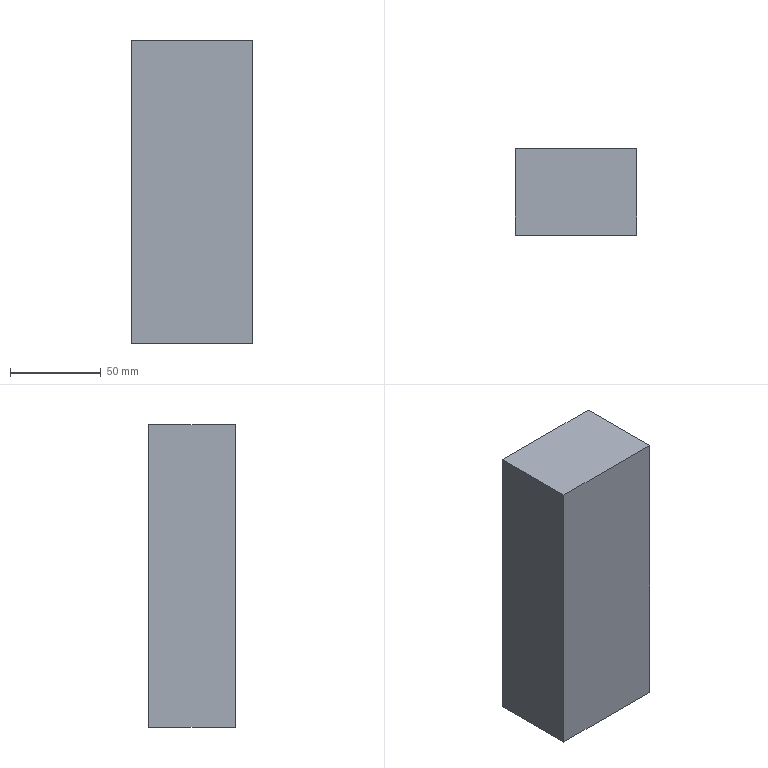Component | SolidWorks | BearingHousingBasePlate-1 | 1 solid | 12 faces | box 67.1 x 48 x 167 mm | volume 344010 mm3 | plane 12 | material 45
STEP:
#1=CARTESIAN_POINT('',(-12.931,-2.058,45.098));
#2=VERTEX_POINT('',#1);
#3=CARTESIAN_POINT('',(-12.931,-3.948,45.098));
#4=VERTEX_POINT('',#3);
#5=CARTESIAN_POINT('',(-12.931,-3.948,45.098));
#6=DIRECTION('',(0.,-1.,-0.));
#7=VECTOR('',#6,39.37);
#8=LINE('',#5,#7);
#9=EDGE_CURVE('',#2,#4,#8,.T.);
#10=ORIENTED_EDGE('',*,*,#9,.T.);
#11=CARTESIAN_POINT('',(-10.29,-3.948,45.098));
#12=VERTEX_POINT('',#11);
#13=CARTESIAN_POINT('',(-10.29,-3.948,45.098));
#14=DIRECTION('',(-1.,0.,-0.));
#15=VECTOR('',#14,39.37);
#16=LINE('',#13,#15);
#17=EDGE_CURVE('',#12,#4,#16,.T.);
#18=ORIENTED_EDGE('',*,*,#17,.F.);
#19=CARTESIAN_POINT('',(-10.29,-2.058,45.098));
#20=VERTEX_POINT('',#19);
#21=CARTESIAN_POINT('',(-10.29,-3.948,45.098));
#22=DIRECTION('',(0.,-1.,-0.));
#23=VECTOR('',#22,39.37);
#24=LINE('',#21,#23);
#25=EDGE_CURVE('',#20,#12,#24,.T.);
#26=ORIENTED_EDGE('',*,*,#25,.F.);
#27=CARTESIAN_POINT('',(-10.29,-2.058,45.098));
#28=DIRECTION('',(-1.,0.,-0.));
#29=VECTOR('',#28,39.37);
#30=LINE('',#27,#29);
#31=EDGE_CURVE('',#20,#2,#30,.T.);
#32=ORIENTED_EDGE('',*,*,#31,.T.);
#33=EDGE_LOOP('',(#10,#18,#26,#32));
#34=FACE_OUTER_BOUND('',#33,.T.);
#35=CARTESIAN_POINT('',(-10.29,-3.948,45.098));
#36=DIRECTION('',(-0.,0.,-1.));
#37=DIRECTION('',(-0.,1.,0.));
#38=AXIS2_PLACEMENT_3D('',#35,#36,#37);
#39=PLANE('',#38);
#40=ADVANCED_FACE('',(#34),#39,.F.);
#41=CARTESIAN_POINT('',(-12.931,-3.948,38.524));
#42=VERTEX_POINT('',#41);
#43=CARTESIAN_POINT('',(-12.931,-3.948,38.524));
#44=DIRECTION('',(-0.,0.,-1.));
#45=VECTOR('',#44,39.37);
#46=LINE('',#43,#45);
#47=EDGE_CURVE('',#4,#42,#46,.T.);
#48=ORIENTED_EDGE('',*,*,#47,.T.);
#49=CARTESIAN_POINT('',(-10.29,-3.948,38.524));
#50=VERTEX_POINT('',#49);
#51=CARTESIAN_POINT('',(-10.29,-3.948,38.524));
#52=DIRECTION('',(-1.,0.,-0.));
#53=VECTOR('',#52,39.37);
#54=LINE('',#51,#53);
#55=EDGE_CURVE('',#50,#42,#54,.T.);
#56=ORIENTED_EDGE('',*,*,#55,.F.);
#57=CARTESIAN_POINT('',(-10.29,-3.948,38.524));
#58=DIRECTION('',(-0.,0.,-1.));
#59=VECTOR('',#58,39.37);
#60=LINE('',#57,#59);
#61=EDGE_CURVE('',#12,#50,#60,.T.);
#62=ORIENTED_EDGE('',*,*,#61,.F.);
#63=ORIENTED_EDGE('',*,*,#17,.T.);
#64=EDGE_LOOP('',(#48,#56,#62,#63));
#65=FACE_OUTER_BOUND('',#64,.T.);
#66=CARTESIAN_POINT('',(-10.29,-3.948,38.524));
#67=DIRECTION('',(-0.,1.,0.));
#68=DIRECTION('',(0.,-0.,1.));
#69=AXIS2_PLACEMENT_3D('',#66,#67,#68);
#70=PLANE('',#69);
#71=ADVANCED_FACE('',(#65),#70,.F.);
#72=CARTESIAN_POINT('',(-12.931,-2.058,38.524));
#73=VERTEX_POINT('',#72);
#74=CARTESIAN_POINT('',(-12.931,-3.948,38.524));
#75=DIRECTION('',(-0.,1.,-0.));
#76=VECTOR('',#75,39.37);
#77=LINE('',#74,#76);
#78=EDGE_CURVE('',#42,#73,#77,.T.);
#79=ORIENTED_EDGE('',*,*,#78,.T.);
#80=CARTESIAN_POINT('',(-10.29,-2.058,38.524));
#81=VERTEX_POINT('',#80);
#82=CARTESIAN_POINT('',(-10.29,-2.058,38.524));
#83=DIRECTION('',(-1.,0.,-0.));
#84=VECTOR('',#83,39.37);
#85=LINE('',#82,#84);
#86=EDGE_CURVE('',#81,#73,#85,.T.);
#87=ORIENTED_EDGE('',*,*,#86,.F.);
#88=CARTESIAN_POINT('',(-10.29,-3.948,38.524));
#89=DIRECTION('',(-0.,1.,-0.));
#90=VECTOR('',#89,39.37);
#91=LINE('',#88,#90);
#92=EDGE_CURVE('',#50,#81,#91,.T.);
#93=ORIENTED_EDGE('',*,*,#92,.F.);
#94=ORIENTED_EDGE('',*,*,#55,.T.);
#95=EDGE_LOOP('',(#79,#87,#93,#94));
#96=FACE_OUTER_BOUND('',#95,.T.);
#97=CARTESIAN_POINT('',(-10.29,-3.948,38.524));
#98=DIRECTION('',(-0.,0.,1.));
#99=DIRECTION('',(1.,-0.,0.));
#100=AXIS2_PLACEMENT_3D('',#97,#98,#99);
#101=PLANE('',#100);
#102=ADVANCED_FACE('',(#96),#101,.F.);
#103=CARTESIAN_POINT('',(-12.931,-2.058,38.524));
#104=DIRECTION('',(0.,0.,1.));
#105=VECTOR('',#104,39.37);
#106=LINE('',#103,#105);
#107=EDGE_CURVE('',#73,#2,#106,.T.);
#108=ORIENTED_EDGE('',*,*,#107,.T.);
#109=ORIENTED_EDGE('',*,*,#31,.F.);
#110=CARTESIAN_POINT('',(-10.29,-2.058,38.524));
#111=DIRECTION('',(0.,0.,1.));
#112=VECTOR('',#111,39.37);
#113=LINE('',#110,#112);
#114=EDGE_CURVE('',#81,#20,#113,.T.);
#115=ORIENTED_EDGE('',*,*,#114,.F.);
#116=ORIENTED_EDGE('',*,*,#86,.T.);
#117=EDGE_LOOP('',(#108,#109,#115,#116));
#118=FACE_OUTER_BOUND('',#117,.T.);
#119=CARTESIAN_POINT('',(-10.29,-2.058,38.524));
#120=DIRECTION('',(0.,-1.,0.));
#121=DIRECTION('',(-0.,-0.,-1.));
#122=AXIS2_PLACEMENT_3D('',#119,#120,#121);
#123=PLANE('',#122);
#124=ADVANCED_FACE('',(#118),#123,.F.);
#125=ORIENTED_EDGE('',*,*,#25,.T.);
#126=ORIENTED_EDGE('',*,*,#61,.T.);
#127=ORIENTED_EDGE('',*,*,#92,.T.);
#128=ORIENTED_EDGE('',*,*,#114,.T.);
#129=EDGE_LOOP('',(#125,#126,#127,#128));
#130=FACE_OUTER_BOUND('',#129,.T.);
#131=CARTESIAN_POINT('',(-10.29,-3.003,41.811));
#132=DIRECTION('',(1.,-0.,-0.));
#133=DIRECTION('',(-0.,-0.,-1.));
#134=AXIS2_PLACEMENT_3D('',#131,#132,#133);
#135=PLANE('',#134);
#136=ADVANCED_FACE('',(#130),#135,.T.);
#137=ORIENTED_EDGE('',*,*,#9,.F.);
#138=ORIENTED_EDGE('',*,*,#107,.F.);
#139=ORIENTED_EDGE('',*,*,#78,.F.);
#140=ORIENTED_EDGE('',*,*,#47,.F.);
#141=EDGE_LOOP('',(#137,#138,#139,#140));
#142=FACE_OUTER_BOUND('',#141,.T.);
#143=CARTESIAN_POINT('',(-12.931,-3.003,41.811));
#144=DIRECTION('',(1.,-0.,-0.));
#145=DIRECTION('',(-0.,-0.,-1.));
#146=AXIS2_PLACEMENT_3D('',#143,#144,#145);
#147=PLANE('',#146);
#148=ADVANCED_FACE('',(#142),#147,.F.);
#149=CLOSED_SHELL('',(#40,#71,#102,#124,#136,#148));
#150=CARTESIAN_POINT('',(-12.538,-2.452,44.705));
#151=VERTEX_POINT('',#150);
#152=CARTESIAN_POINT('',(-12.538,-3.555,44.705));
#153=VERTEX_POINT('',#152);
#154=CARTESIAN_POINT('',(-12.538,-3.948,44.705));
#155=DIRECTION('',(0.,-1.,-0.));
#156=VECTOR('',#155,39.37);
#157=LINE('',#154,#156);
#158=EDGE_CURVE('',#151,#153,#157,.T.);
#159=ORIENTED_EDGE('',*,*,#158,.F.);
#160=CARTESIAN_POINT('',(-10.683,-2.452,44.705));
#161=VERTEX_POINT('',#160);
#162=CARTESIAN_POINT('',(-10.683,-2.452,44.705));
#163=DIRECTION('',(-1.,0.,-0.));
#164=VECTOR('',#163,39.37);
#165=LINE('',#162,#164);
#166=EDGE_CURVE('',#161,#151,#165,.T.);
#167=ORIENTED_EDGE('',*,*,#166,.F.);
#168=CARTESIAN_POINT('',(-10.683,-3.555,44.705));
#169=VERTEX_POINT('',#168);
#170=CARTESIAN_POINT('',(-10.683,-3.948,44.705));
#171=DIRECTION('',(0.,-1.,-0.));
#172=VECTOR('',#171,39.37);
#173=LINE('',#170,#172);
#174=EDGE_CURVE('',#161,#169,#173,.T.);
#175=ORIENTED_EDGE('',*,*,#174,.T.);
#176=CARTESIAN_POINT('',(-10.683,-3.555,44.705));
#177=DIRECTION('',(-1.,0.,-0.));
#178=VECTOR('',#177,39.37);
#179=LINE('',#176,#178);
#180=EDGE_CURVE('',#169,#153,#179,.T.);
#181=ORIENTED_EDGE('',*,*,#180,.T.);
#182=EDGE_LOOP('',(#159,#167,#175,#181));
#183=FACE_OUTER_BOUND('',#182,.T.);
#184=CARTESIAN_POINT('',(-10.683,-3.948,44.705));
#185=DIRECTION('',(-0.,0.,-1.));
#186=DIRECTION('',(-0.,1.,0.));
#187=AXIS2_PLACEMENT_3D('',#184,#185,#186);
#188=PLANE('',#187);
#189=ADVANCED_FACE('',(#183),#188,.T.);
#190=CARTESIAN_POINT('',(-12.538,-3.555,38.917));
#191=VERTEX_POINT('',#190);
#192=CARTESIAN_POINT('',(-12.538,-3.555,38.524));
#193=DIRECTION('',(-0.,0.,-1.));
#194=VECTOR('',#193,39.37);
#195=LINE('',#192,#194);
#196=EDGE_CURVE('',#153,#191,#195,.T.);
#197=ORIENTED_EDGE('',*,*,#196,.F.);
#198=ORIENTED_EDGE('',*,*,#180,.F.);
#199=CARTESIAN_POINT('',(-10.683,-3.555,38.917));
#200=VERTEX_POINT('',#199);
#201=CARTESIAN_POINT('',(-10.683,-3.555,38.524));
#202=DIRECTION('',(-0.,0.,-1.));
#203=VECTOR('',#202,39.37);
#204=LINE('',#201,#203);
#205=EDGE_CURVE('',#169,#200,#204,.T.);
#206=ORIENTED_EDGE('',*,*,#205,.T.);
#207=CARTESIAN_POINT('',(-10.683,-3.555,38.917));
#208=DIRECTION('',(-1.,0.,-0.));
#209=VECTOR('',#208,39.37);
#210=LINE('',#207,#209);
#211=EDGE_CURVE('',#200,#191,#210,.T.);
#212=ORIENTED_EDGE('',*,*,#211,.T.);
#213=EDGE_LOOP('',(#197,#198,#206,#212));
#214=FACE_OUTER_BOUND('',#213,.T.);
#215=CARTESIAN_POINT('',(-10.683,-3.555,38.524));
#216=DIRECTION('',(-0.,1.,0.));
#217=DIRECTION('',(0.,-0.,1.));
#218=AXIS2_PLACEMENT_3D('',#215,#216,#217);
#219=PLANE('',#218);
#220=ADVANCED_FACE('',(#214),#219,.T.);
#221=CARTESIAN_POINT('',(-12.538,-2.452,38.917));
#222=VERTEX_POINT('',#221);
#223=CARTESIAN_POINT('',(-12.538,-3.948,38.917));
#224=DIRECTION('',(-0.,1.,-0.));
#225=VECTOR('',#224,39.37);
#226=LINE('',#223,#225);
#227=EDGE_CURVE('',#191,#222,#226,.T.);
#228=ORIENTED_EDGE('',*,*,#227,.F.);
#229=ORIENTED_EDGE('',*,*,#211,.F.);
#230=CARTESIAN_POINT('',(-10.683,-2.452,38.917));
#231=VERTEX_POINT('',#230);
#232=CARTESIAN_POINT('',(-10.683,-3.948,38.917));
#233=DIRECTION('',(-0.,1.,-0.));
#234=VECTOR('',#233,39.37);
#235=LINE('',#232,#234);
#236=EDGE_CURVE('',#200,#231,#235,.T.);
#237=ORIENTED_EDGE('',*,*,#236,.T.);
#238=CARTESIAN_POINT('',(-10.683,-2.452,38.917));
#239=DIRECTION('',(-1.,0.,-0.));
#240=VECTOR('',#239,39.37);
#241=LINE('',#238,#240);
#242=EDGE_CURVE('',#231,#222,#241,.T.);
#243=ORIENTED_EDGE('',*,*,#242,.T.);
#244=EDGE_LOOP('',(#228,#229,#237,#243));
#245=FACE_OUTER_BOUND('',#244,.T.);
#246=CARTESIAN_POINT('',(-10.683,-3.948,38.917));
#247=DIRECTION('',(-0.,0.,1.));
#248=DIRECTION('',(1.,-0.,0.));
#249=AXIS2_PLACEMENT_3D('',#246,#247,#248);
#250=PLANE('',#249);
#251=ADVANCED_FACE('',(#245),#250,.T.);
#252=CARTESIAN_POINT('',(-12.538,-2.452,38.524));
#253=DIRECTION('',(0.,0.,1.));
#254=VECTOR('',#253,39.37);
#255=LINE('',#252,#254);
#256=EDGE_CURVE('',#222,#151,#255,.T.);
#257=ORIENTED_EDGE('',*,*,#256,.F.);
#258=ORIENTED_EDGE('',*,*,#242,.F.);
#259=CARTESIAN_POINT('',(-10.683,-2.452,38.524));
#260=DIRECTION('',(0.,0.,1.));
#261=VECTOR('',#260,39.37);
#262=LINE('',#259,#261);
#263=EDGE_CURVE('',#231,#161,#262,.T.);
#264=ORIENTED_EDGE('',*,*,#263,.T.);
#265=ORIENTED_EDGE('',*,*,#166,.T.);
#266=EDGE_LOOP('',(#257,#258,#264,#265));
#267=FACE_OUTER_BOUND('',#266,.T.);
#268=CARTESIAN_POINT('',(-10.683,-2.452,38.524));
#269=DIRECTION('',(0.,-1.,0.));
#270=DIRECTION('',(-0.,-0.,-1.));
#271=AXIS2_PLACEMENT_3D('',#268,#269,#270);
#272=PLANE('',#271);
#273=ADVANCED_FACE('',(#267),#272,.T.);
#274=ORIENTED_EDGE('',*,*,#174,.F.);
#275=ORIENTED_EDGE('',*,*,#263,.F.);
#276=ORIENTED_EDGE('',*,*,#236,.F.);
#277=ORIENTED_EDGE('',*,*,#205,.F.);
#278=EDGE_LOOP('',(#274,#275,#276,#277));
#279=FACE_OUTER_BOUND('',#278,.T.);
#280=CARTESIAN_POINT('',(-10.683,-3.003,41.811));
#281=DIRECTION('',(1.,-0.,-0.));
#282=DIRECTION('',(-0.,-0.,-1.));
#283=AXIS2_PLACEMENT_3D('',#280,#281,#282);
#284=PLANE('',#283);
#285=ADVANCED_FACE('',(#279),#284,.F.);
#286=ORIENTED_EDGE('',*,*,#158,.T.);
#287=ORIENTED_EDGE('',*,*,#196,.T.);
#288=ORIENTED_EDGE('',*,*,#227,.T.);
#289=ORIENTED_EDGE('',*,*,#256,.T.);
#290=EDGE_LOOP('',(#286,#287,#288,#289));
#291=FACE_OUTER_BOUND('',#290,.T.);
#292=CARTESIAN_POINT('',(-12.538,-3.003,41.811));
#293=DIRECTION('',(1.,-0.,-0.));
#294=DIRECTION('',(-0.,-0.,-1.));
#295=AXIS2_PLACEMENT_3D('',#292,#293,#294);
#296=PLANE('',#295);
#297=ADVANCED_FACE('',(#291),#296,.T.);
#298=CLOSED_SHELL('',(#189,#220,#251,#273,#285,#297));
#299=ORIENTED_CLOSED_SHELL('',*,#298,.F.);
#300=BREP_WITH_VOIDS('',#149,(#299));
#301=CARTESIAN_POINT('',(0.,0.,0.));
#302=DIRECTION('',(0.,0.,1.));
#303=DIRECTION('',(1.,0.,0.));
#304=AXIS2_PLACEMENT_3D('',#301,#302,#303);
#305=(LENGTH_UNIT()NAMED_UNIT(*)SI_UNIT($,.METRE.));
#306=LENGTH_MEASURE_WITH_UNIT(LENGTH_MEASURE(0.0254),#305);
#307=DIMENSIONAL_EXPONENTS(1.,0.,0.,0.,0.,0.,0.);
#308=(CONVERSION_BASED_UNIT('',#306)LENGTH_UNIT()NAMED_UNIT(#307));
#309=UNCERTAINTY_MEASURE_WITH_UNIT(LENGTH_MEASURE(0.00001),#308,'','');
#310=(NAMED_UNIT(*)PLANE_ANGLE_UNIT()SI_UNIT($,.RADIAN.));
#311=(NAMED_UNIT(*)SI_UNIT($,.STERADIAN.)SOLID_ANGLE_UNIT());
#312=(GEOMETRIC_REPRESENTATION_CONTEXT(3)GLOBAL_UNCERTAINTY_ASSIGNED_CONTEXT((#309))GLOBAL_UNIT_ASSIGNED_CONTEXT((#308,#310,#311))REPRESENTATION_CONTEXT('',''));
#313=ADVANCED_BREP_SHAPE_REPRESENTATION('',(#300,#304),#312);
#314=COLOUR_RGB('',0.7922,0.8196,0.9333);
#315=FILL_AREA_STYLE_COLOUR('',#314);
#316=FILL_AREA_STYLE('',(#315));
#317=SURFACE_STYLE_FILL_AREA(#316);
#318=SURFACE_SIDE_STYLE('',(#317));
#319=SURFACE_STYLE_USAGE(.BOTH.,#318);
#320=PRESENTATION_STYLE_ASSIGNMENT((#319));
#321=STYLED_ITEM('',(#320),#300);
#322=PRESENTATION_LAYER_ASSIGNMENT('','',(#321));
#323=(LENGTH_UNIT()NAMED_UNIT(*)SI_UNIT($,.METRE.));
#324=LENGTH_MEASURE_WITH_UNIT(LENGTH_MEASURE(0.0254),#323);
#325=DIMENSIONAL_EXPONENTS(1.,0.,0.,0.,0.,0.,0.);
#326=(CONVERSION_BASED_UNIT('',#324)LENGTH_UNIT()NAMED_UNIT(#325));
#327=UNCERTAINTY_MEASURE_WITH_UNIT(LENGTH_MEASURE(0.00001),#326,'','');
#328=(NAMED_UNIT(*)PLANE_ANGLE_UNIT()SI_UNIT($,.RADIAN.));
#329=(NAMED_UNIT(*)SI_UNIT($,.STERADIAN.)SOLID_ANGLE_UNIT());
#330=(GEOMETRIC_REPRESENTATION_CONTEXT(3)GLOBAL_UNCERTAINTY_ASSIGNED_CONTEXT((#327))GLOBAL_UNIT_ASSIGNED_CONTEXT((#326,#328,#329))REPRESENTATION_CONTEXT('',''));
#331=MECHANICAL_DESIGN_GEOMETRIC_PRESENTATION_REPRESENTATION('',(#321),#330);